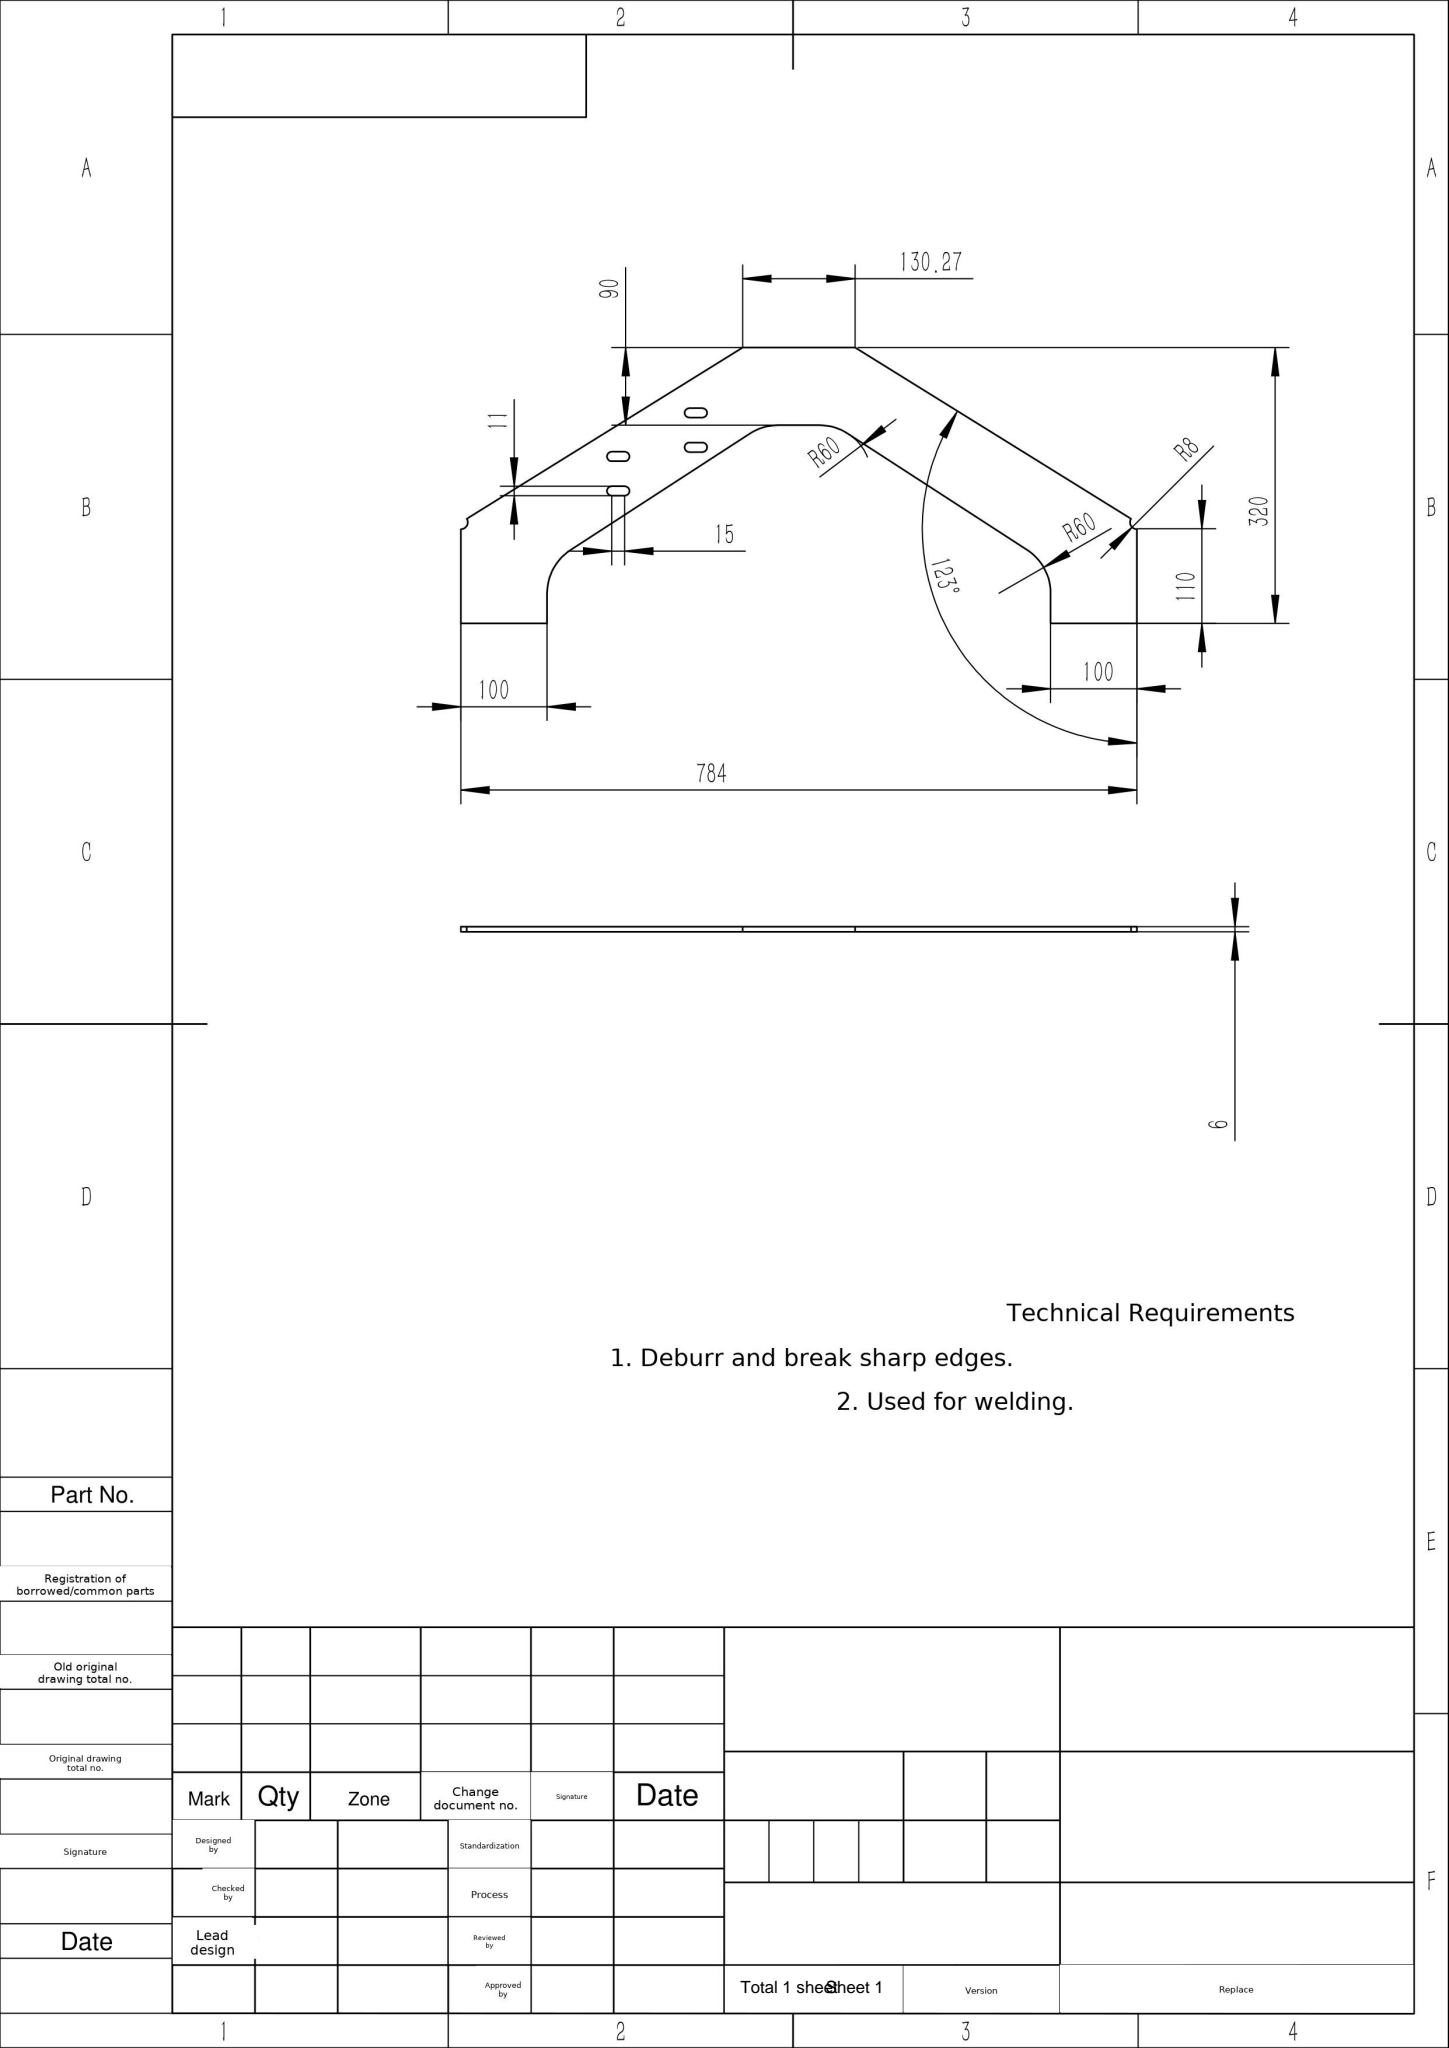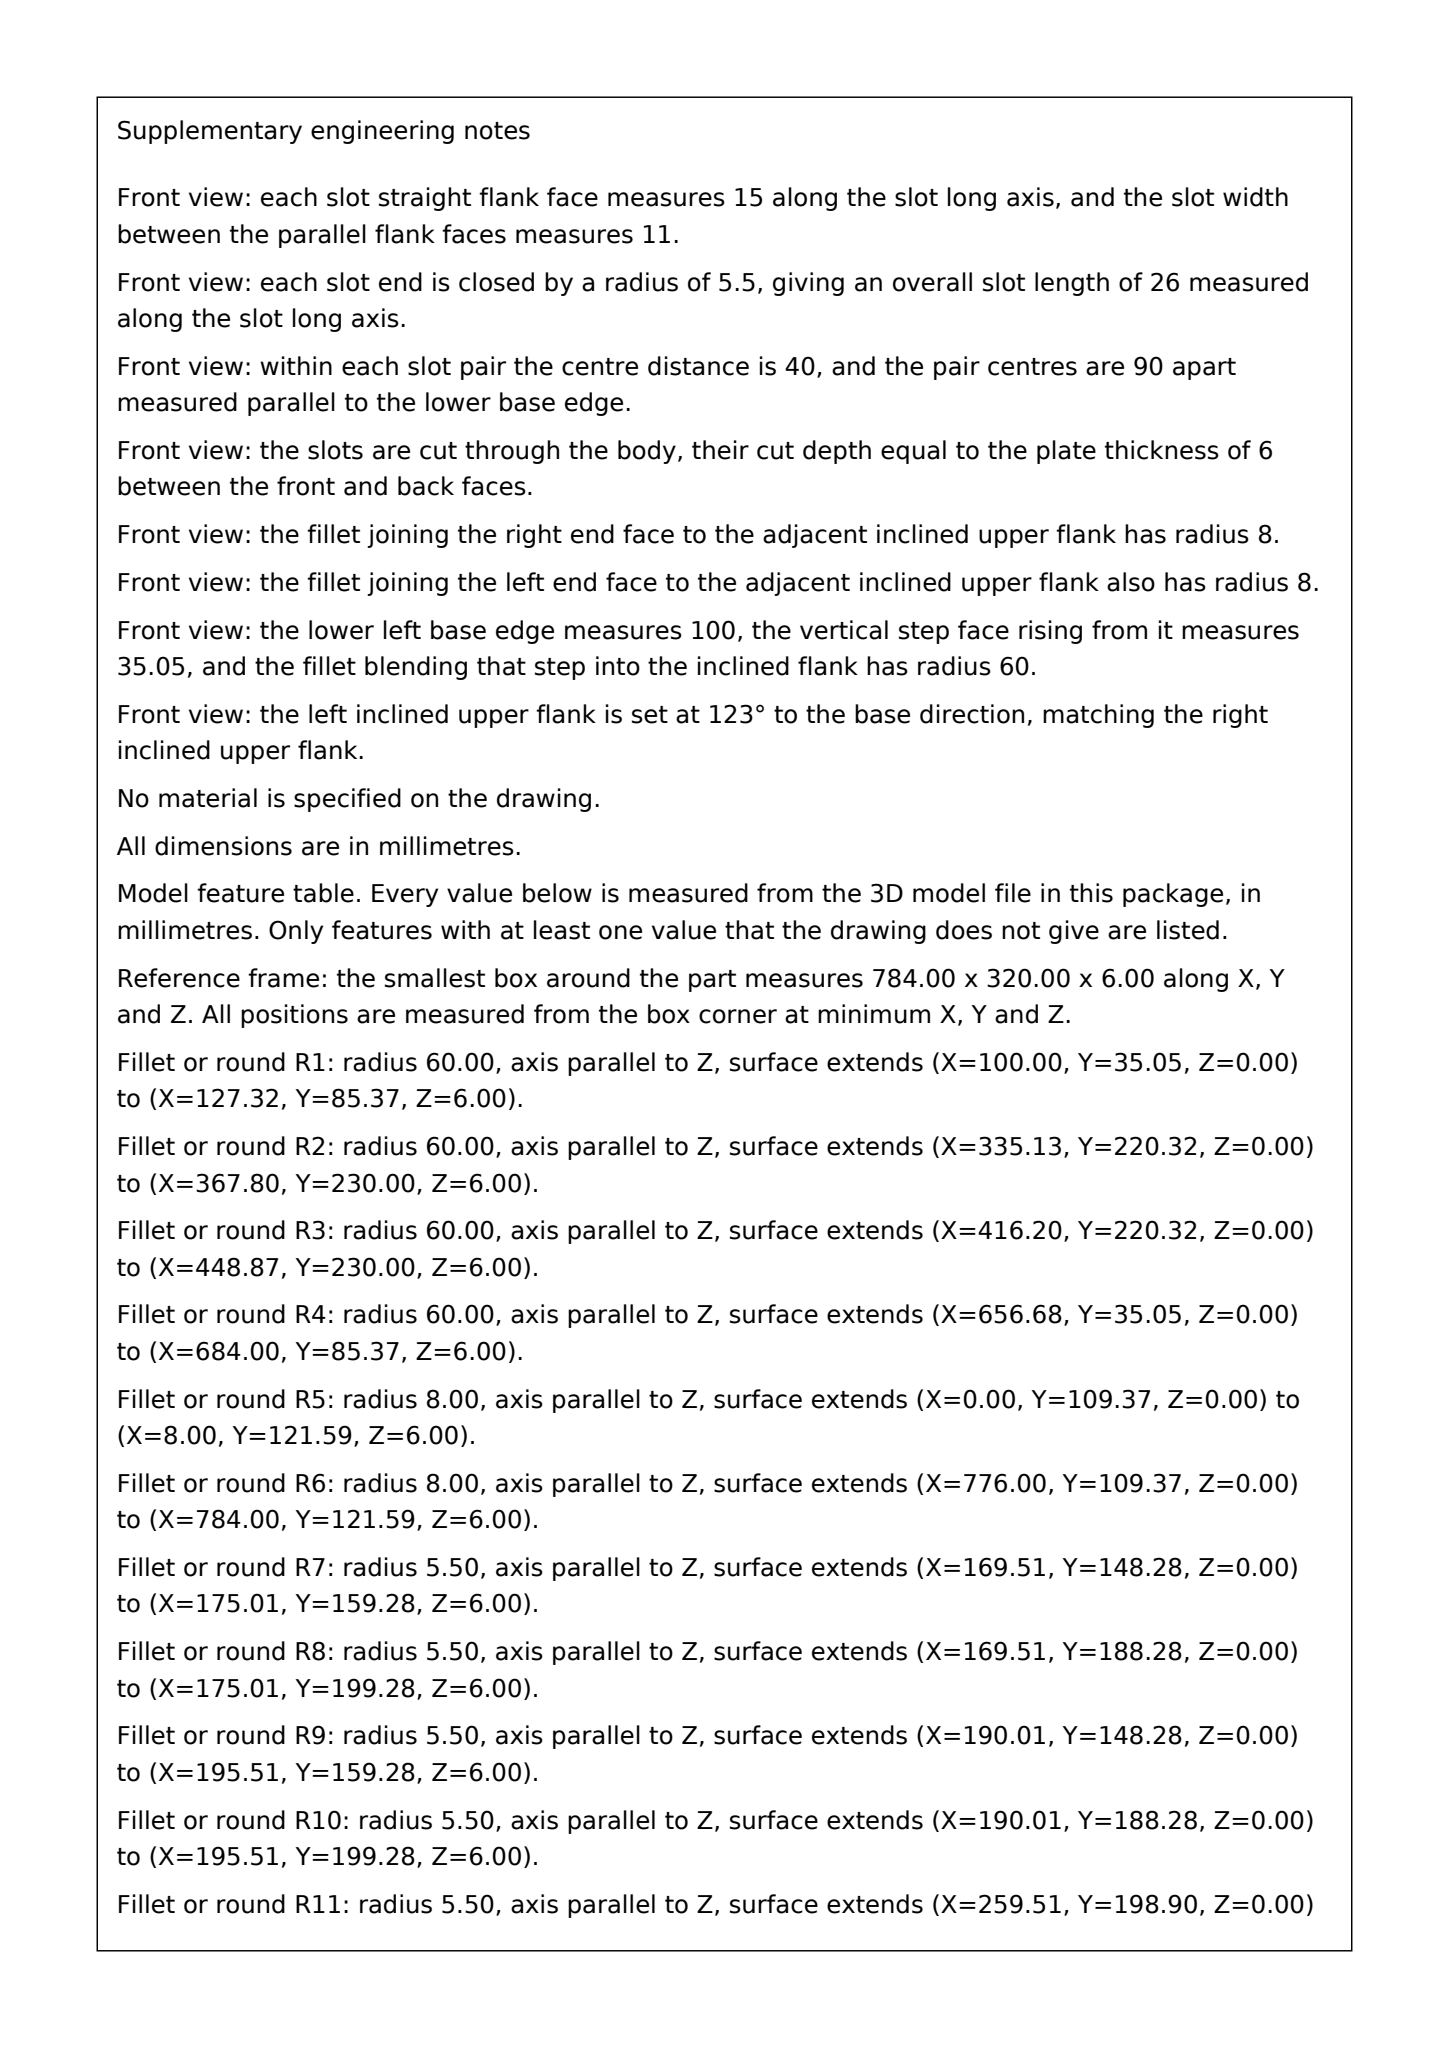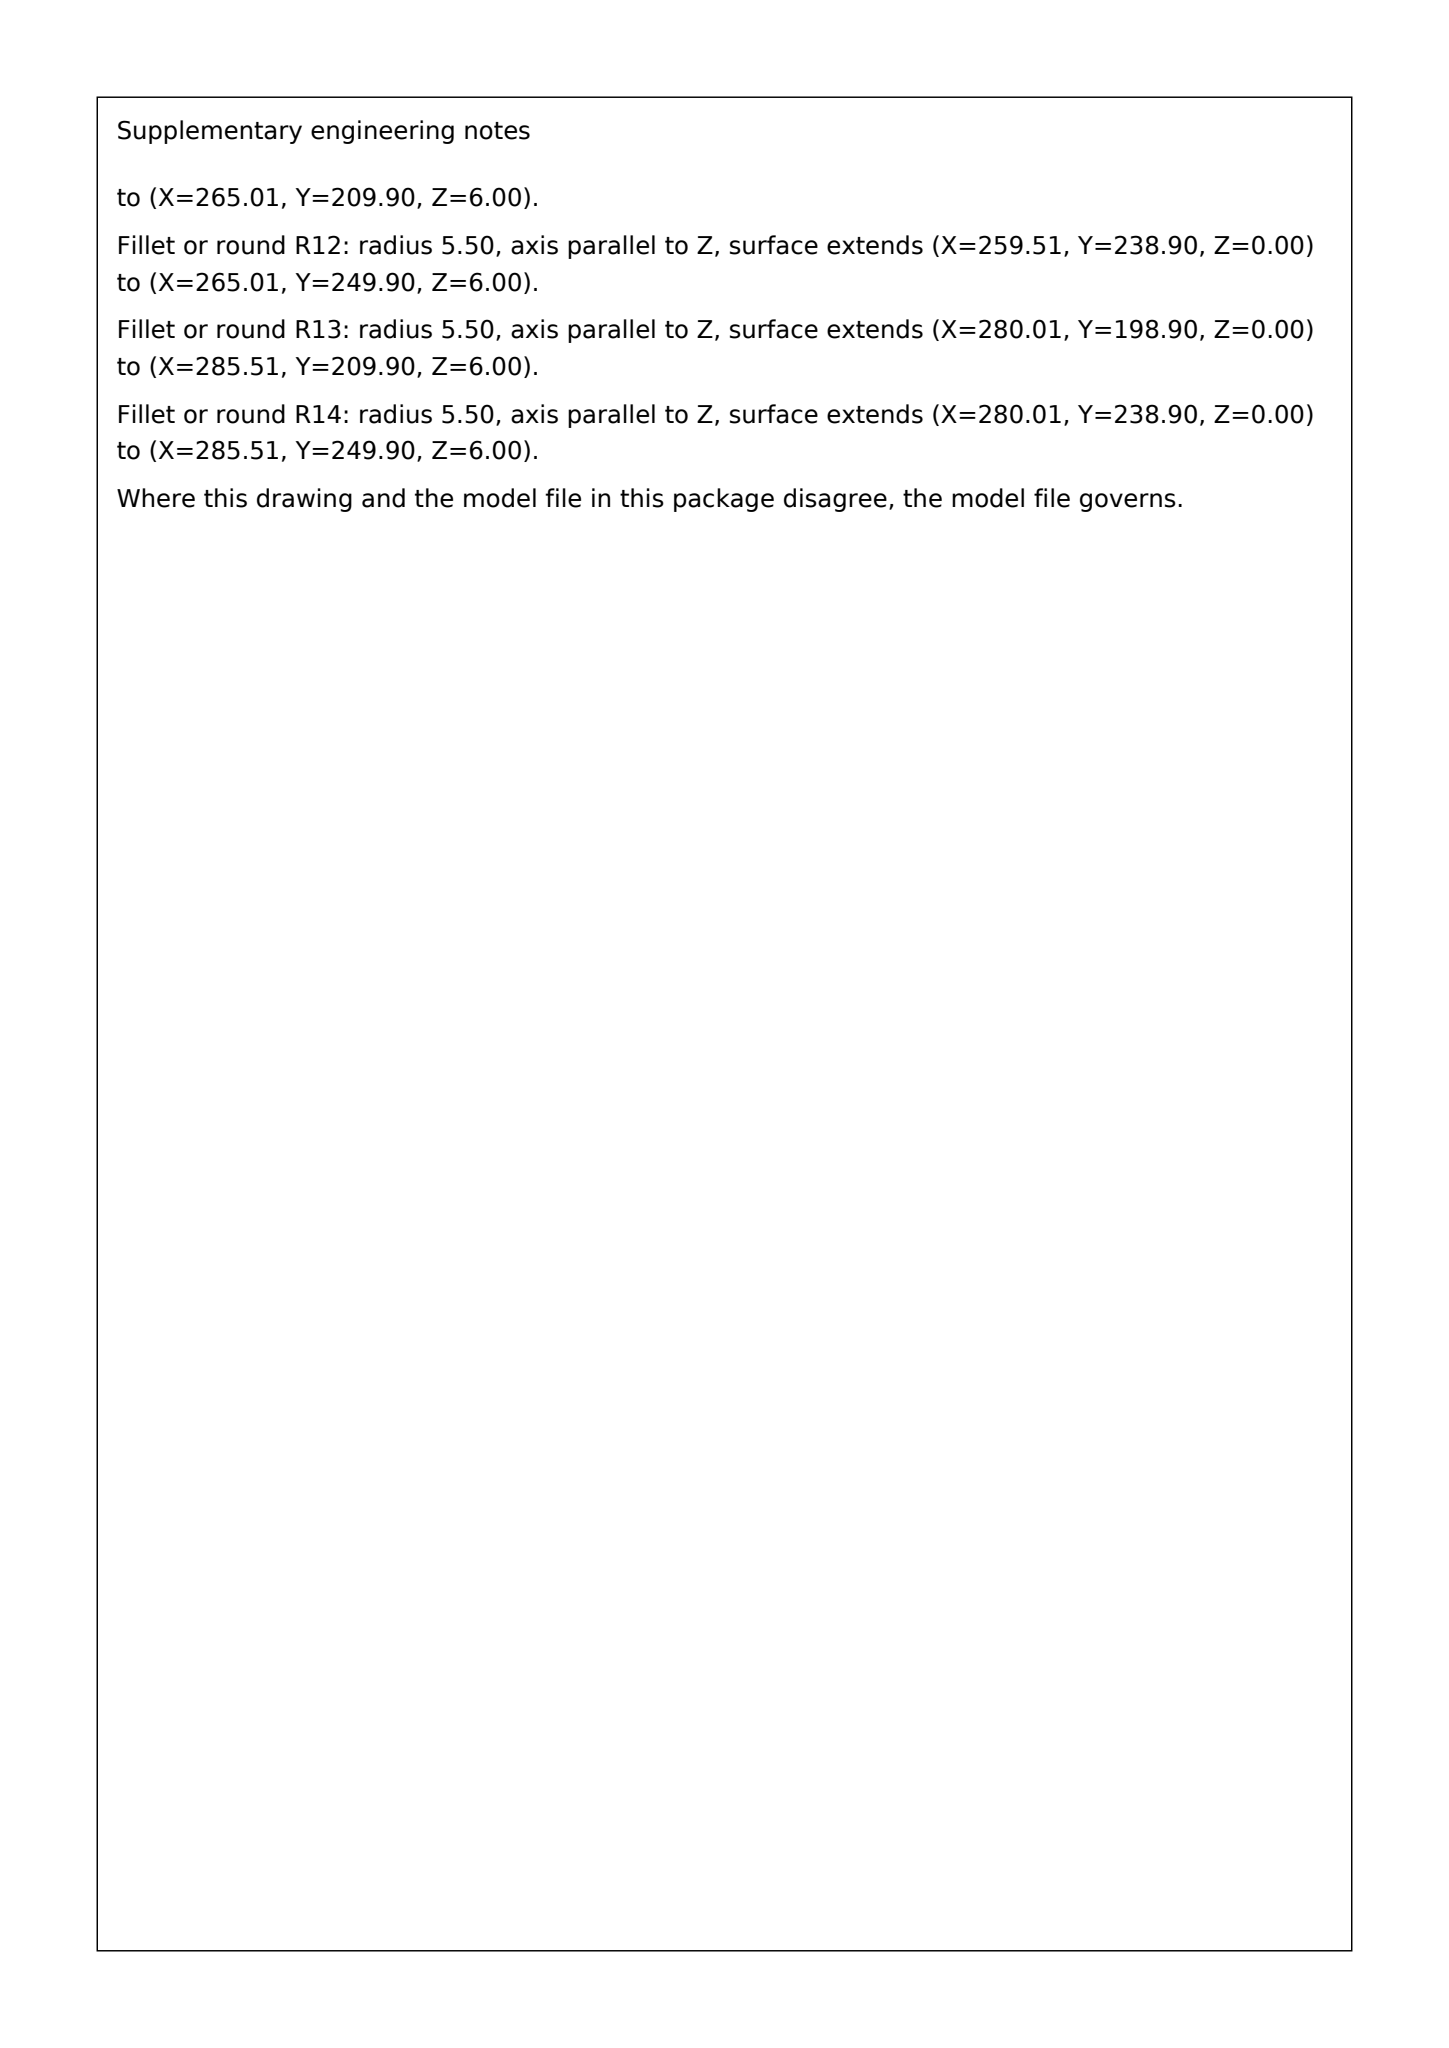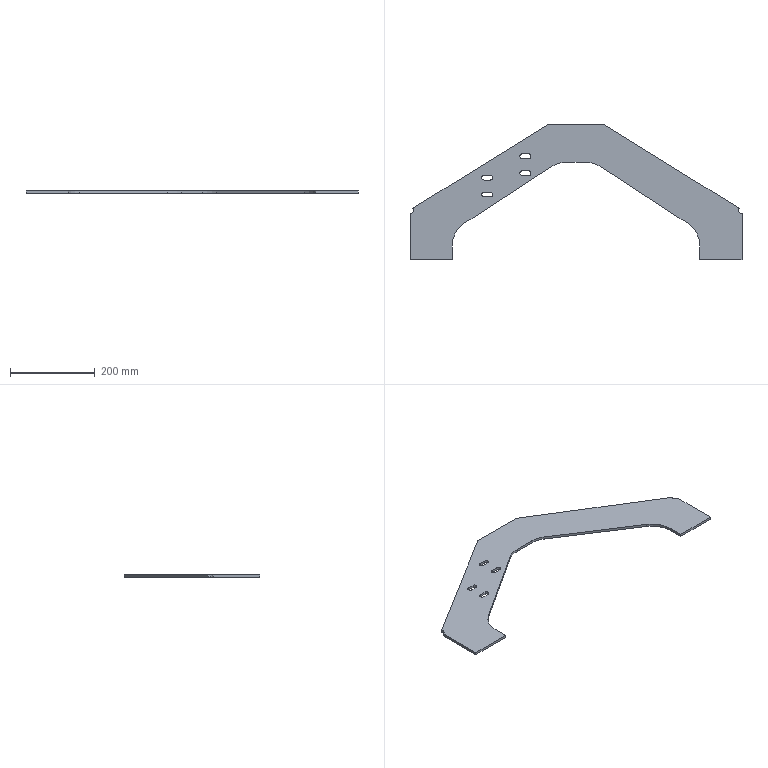Part | SolidWorks | mm | 1 solid | 41 faces | box 784 x 320 x 6 mm | volume 540821 mm3 | plane 22 | cylinder 19 | commonest cylinder face diameters 11 x12 120 x4 16 x3
Drawing notes:
4X SLOT 11W,15 C/C: X175/265, Y153.8&193.8 / 204.4&244.4 FR LL CNR | from the solid: Ø11 z-cyls at (175.01,153.78),(190.01,153.78),(175.01,193.78),(190.01,193.78) and (265.01,204.4),(280.01,204.4),(265.01,244.4),(280.01,244.4); 40 Y spacing, 15 C/C length, bbox 784x320
2X Ø16 HALF-RD NOTCH AT X0 & X784 EDGES, Y117.37 FR BTM EDGE | from the solid: Ø16 z-cyls at (0.0,117.37) and (784.0,117.37), len 6; x planes 0.0 and 784.0
OUTLINE SYM ABOUT PART CL: LH EDGE 123°, LH END FACE 110 HIGH | from the solid: Planes x=0/x=100 mirror x=684/x=784; Ø16 at (0,117.37) and (784,117.37); y=0..110 end faces; bbox 784 wide
130.27 TOP PLATEAU CTRD ON PART CL, 326.87 FROM LH END FACE | from the solid: Top plane y=320; plateau 130.27 wide centred at x=392 (=784/2), per R60 crown centres x=367.8/416.2 midpoint 392
48.4 FLAT AT ARCH CROWN (Y=230) BTWN R60s, CTRD ON PART CL | from the solid: Plane y=230 = 170+60; R60 crown centres x=367.8 and 416.2 -> flat 48.4 lg, midpoint x=392
R60 TYP 4 PLCS (2 ARCH CROWN, 2 LEG ROOT) | from the solid: Ø120 (R60) cyls at (367.8,170), (416.2,170), (160,35.05), (624,35.05)
INNER SLOPED EDGE OF EACH ARM IS TANGENT TO BOTH R60s: LEG-ROOT R60 CTR AT X160, Y35.05 AND ARCH-CROWN R60 CTR AT X367.8, Y170 FROM LL CNR (MIRRORED: X624, Y35.05 AND X416.2, Y170); EDGE RUNS AT 33° TO BTM EDGE | from the solid: cylinders dia 120 (R60) axis z at [160,35.05], [367.8,170], [416.2,170], [624,35.05]